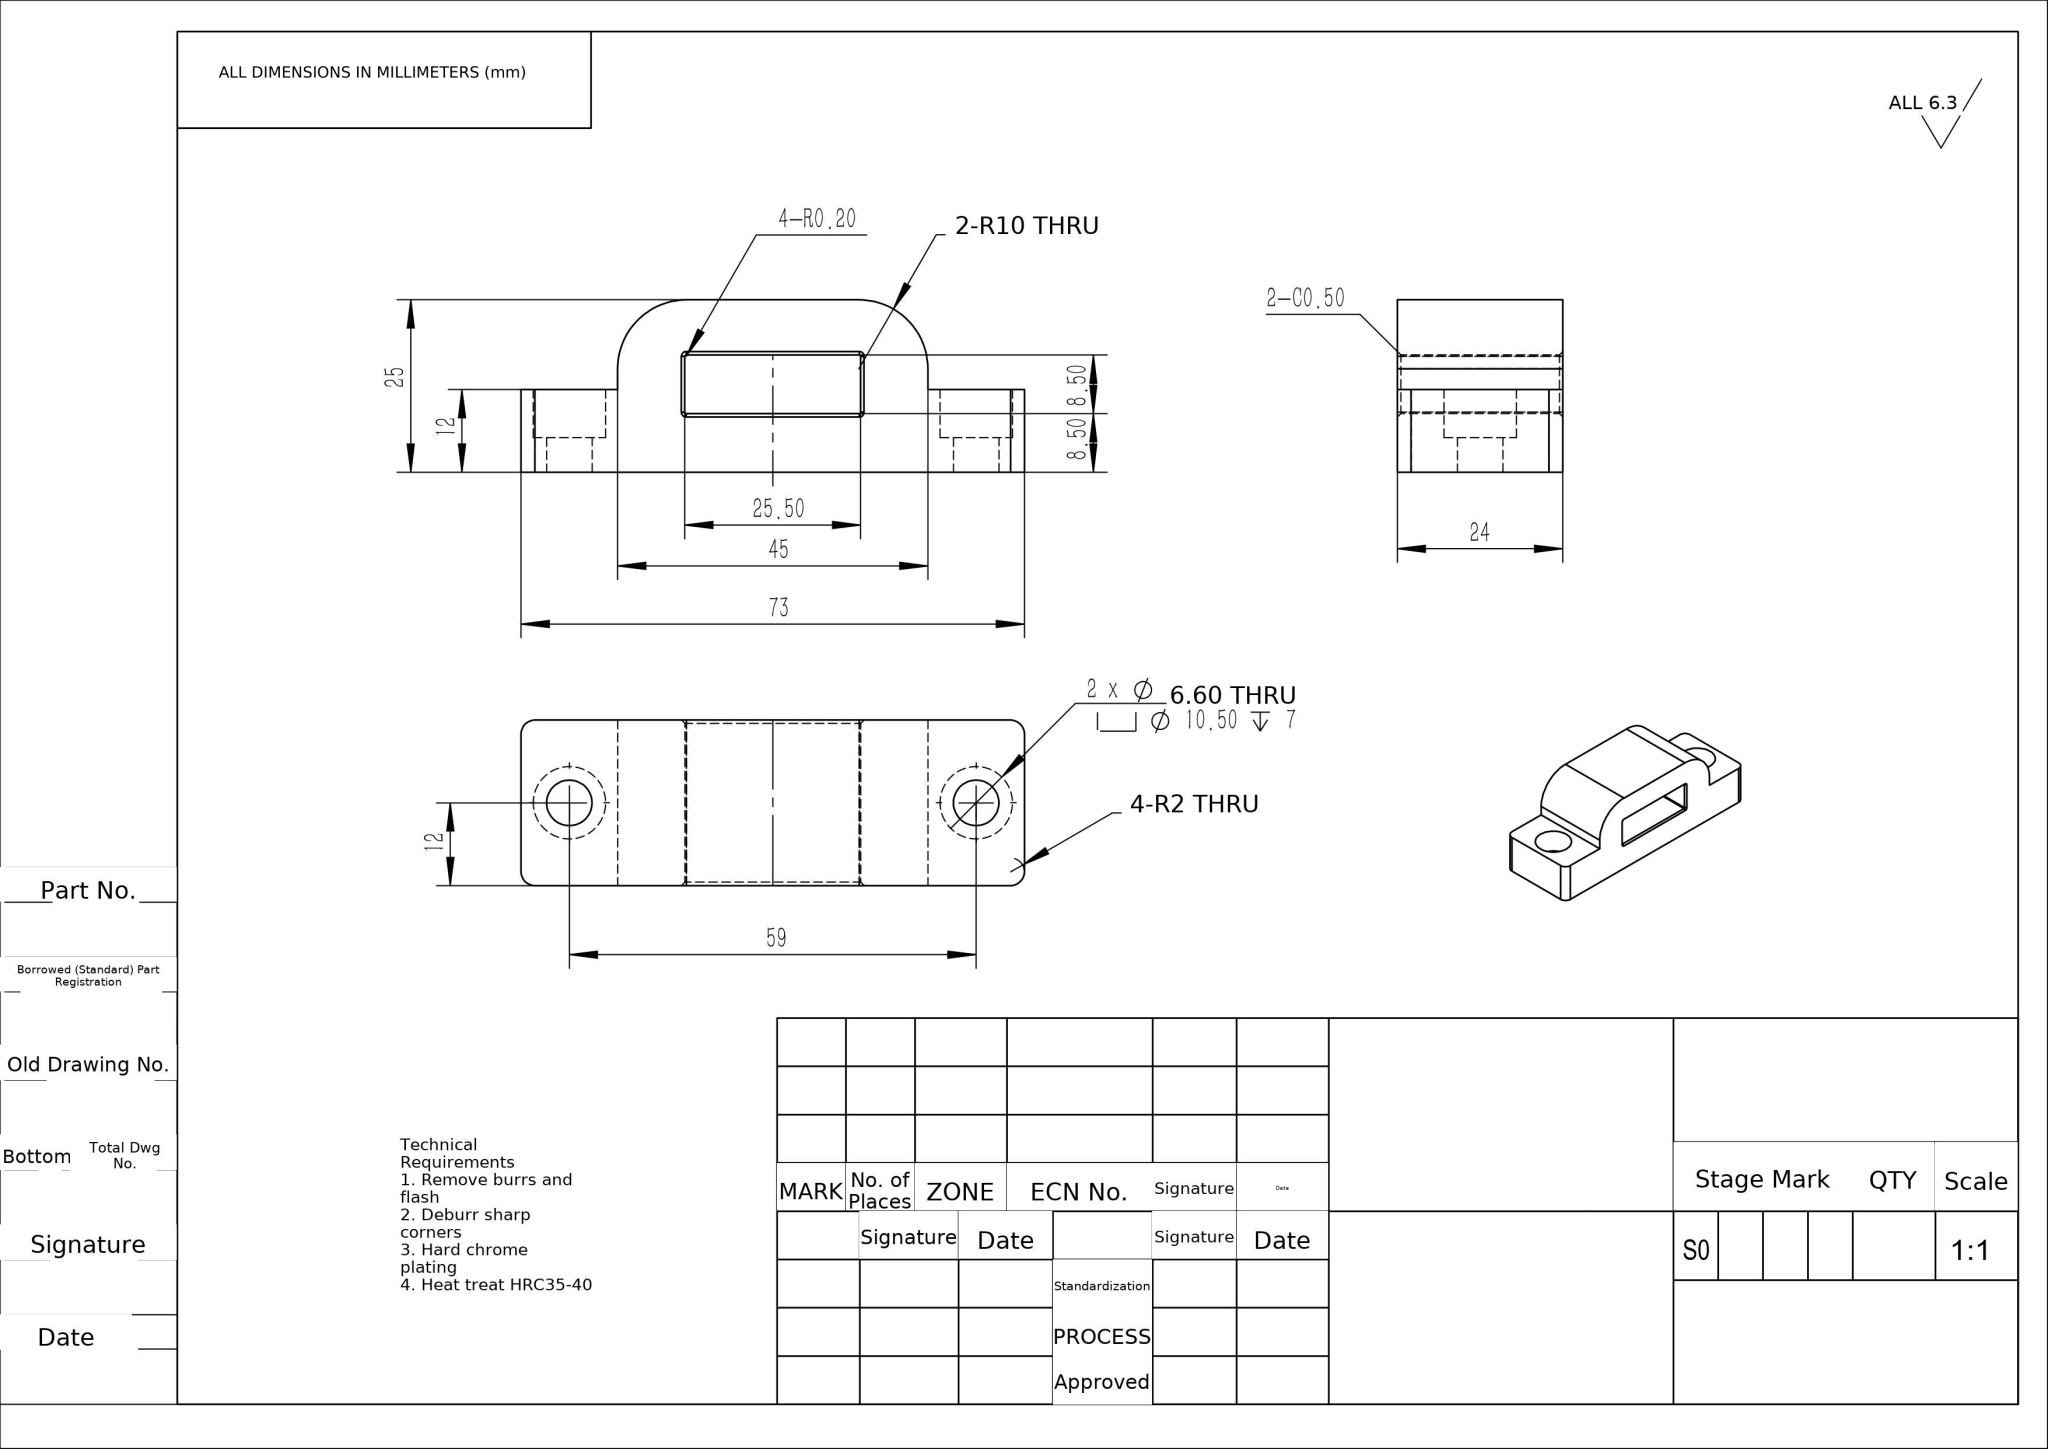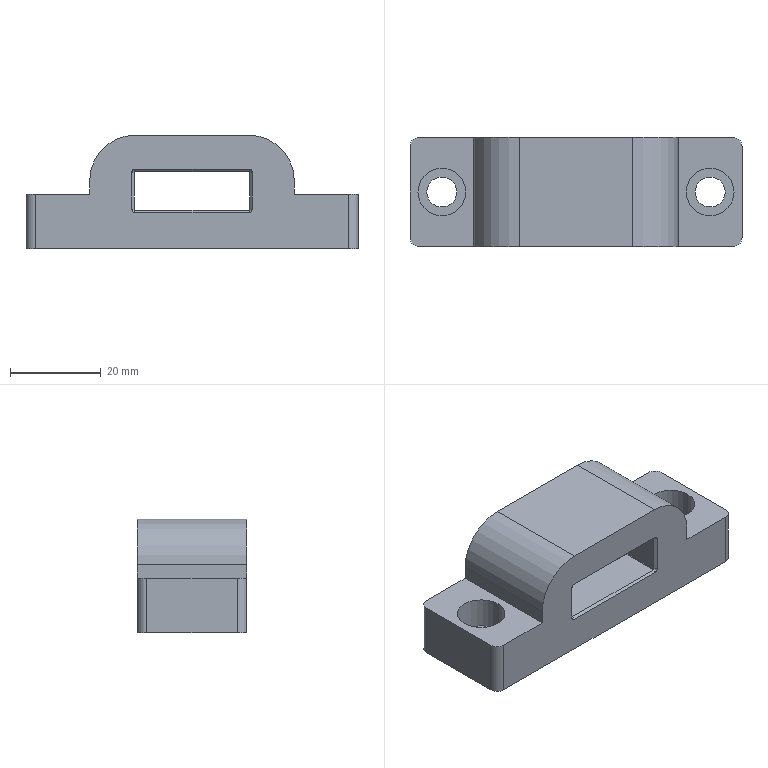Part | NX | mm | 1 solid | 50 faces | box 73 x 24 x 25 mm | volume 27220 mm3 | plane 24 | cylinder 18 | cone 8 | commonest cylinder face diameters 10.5 x4 6.6 x4 0.4 x4 4 x4 20 x2